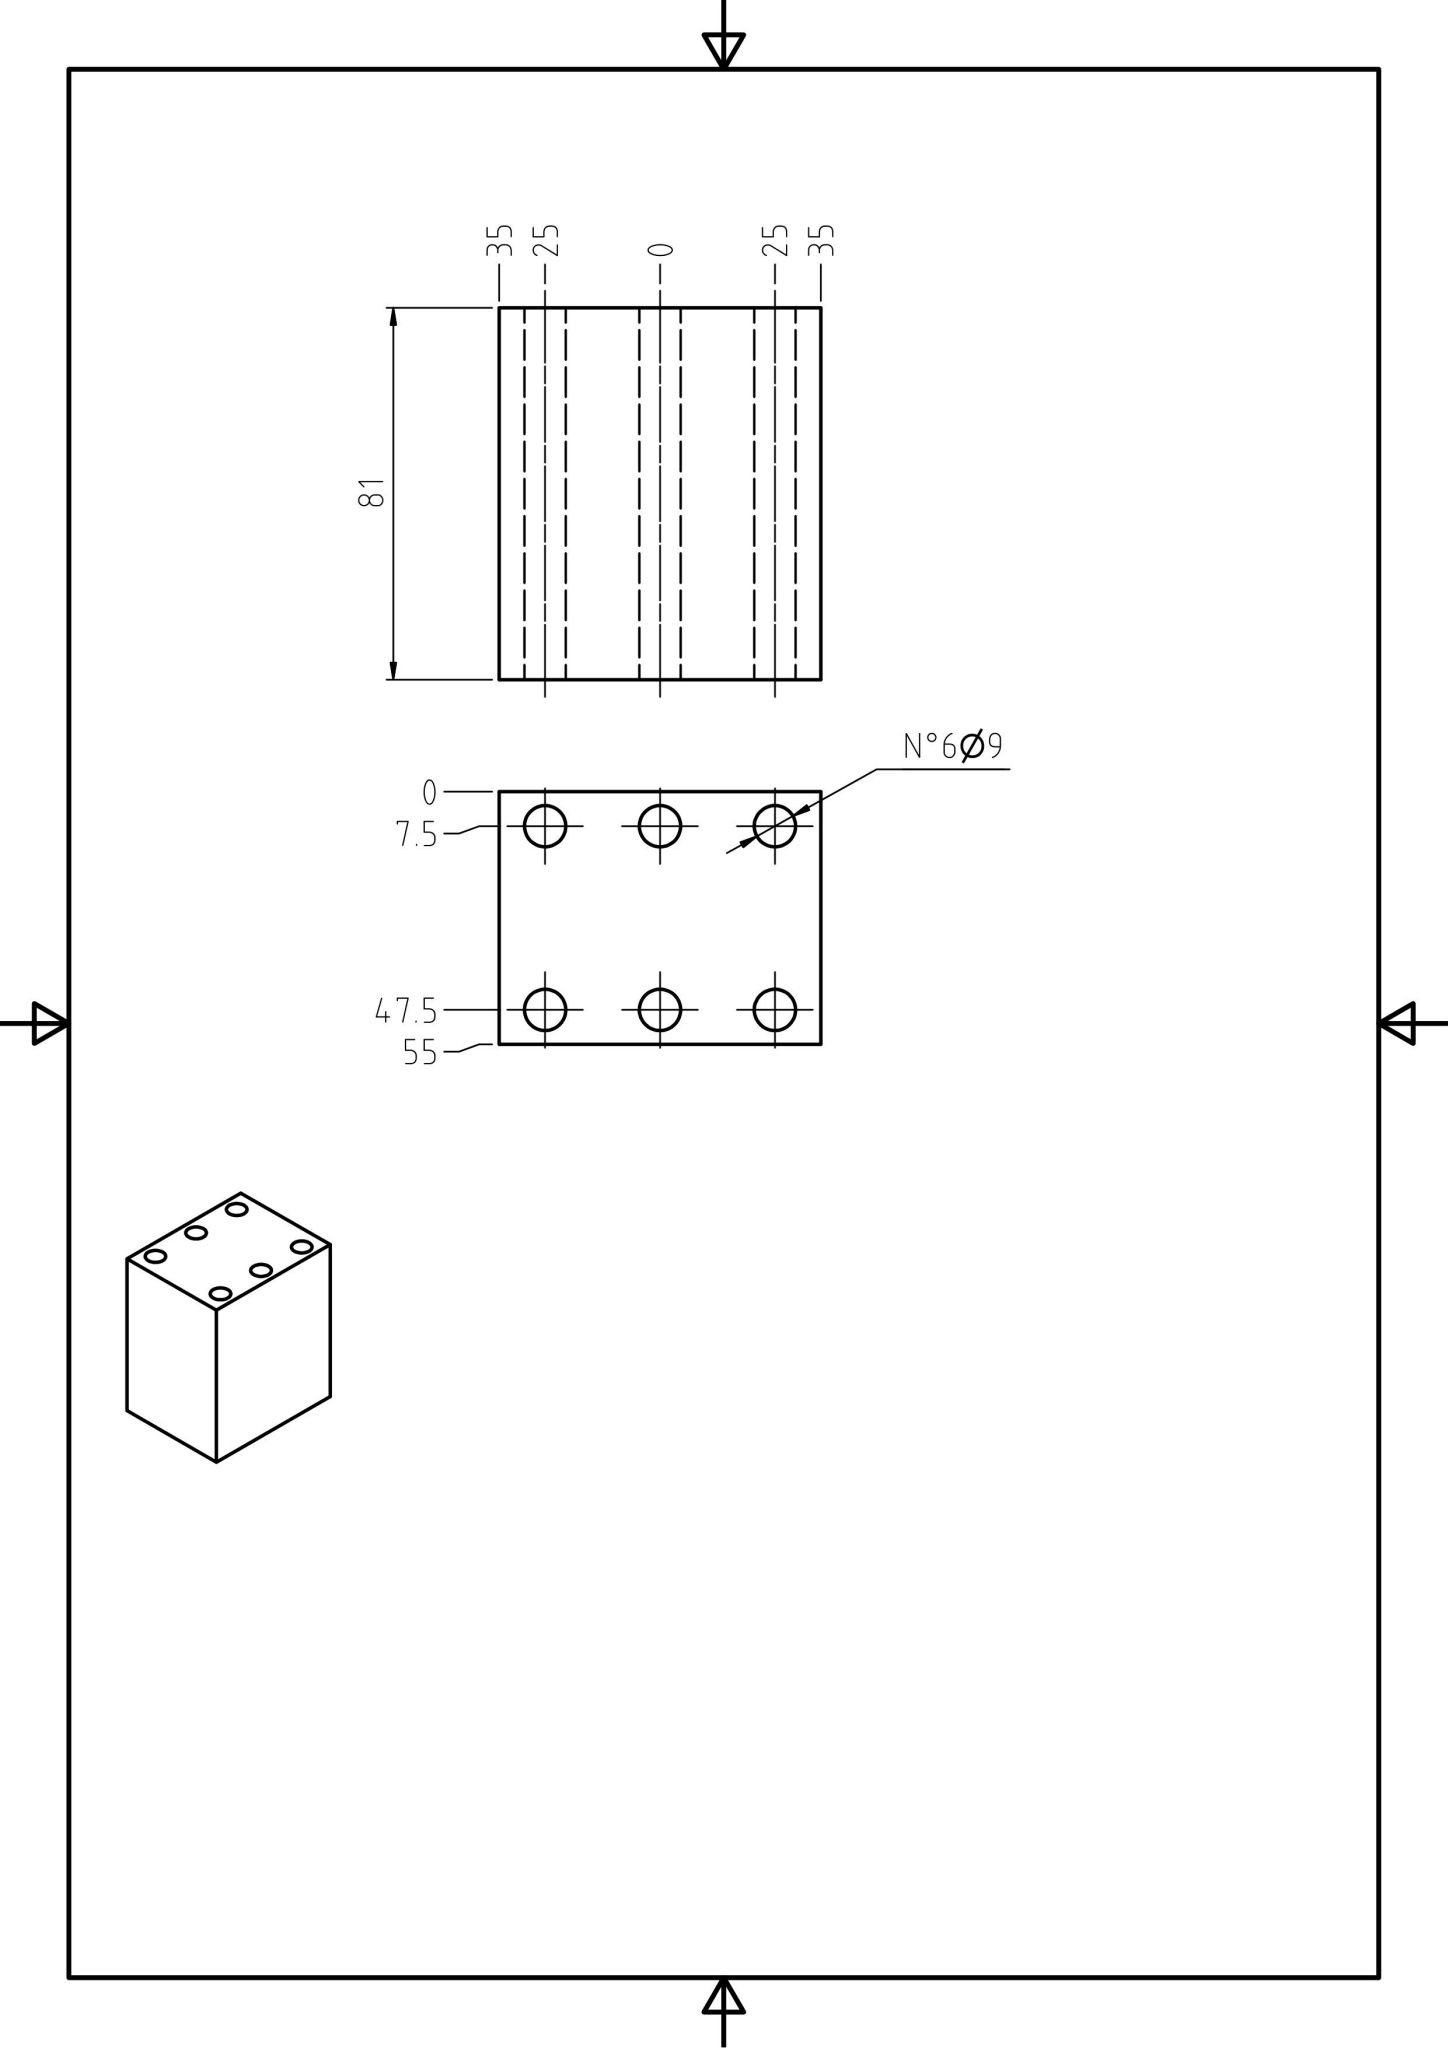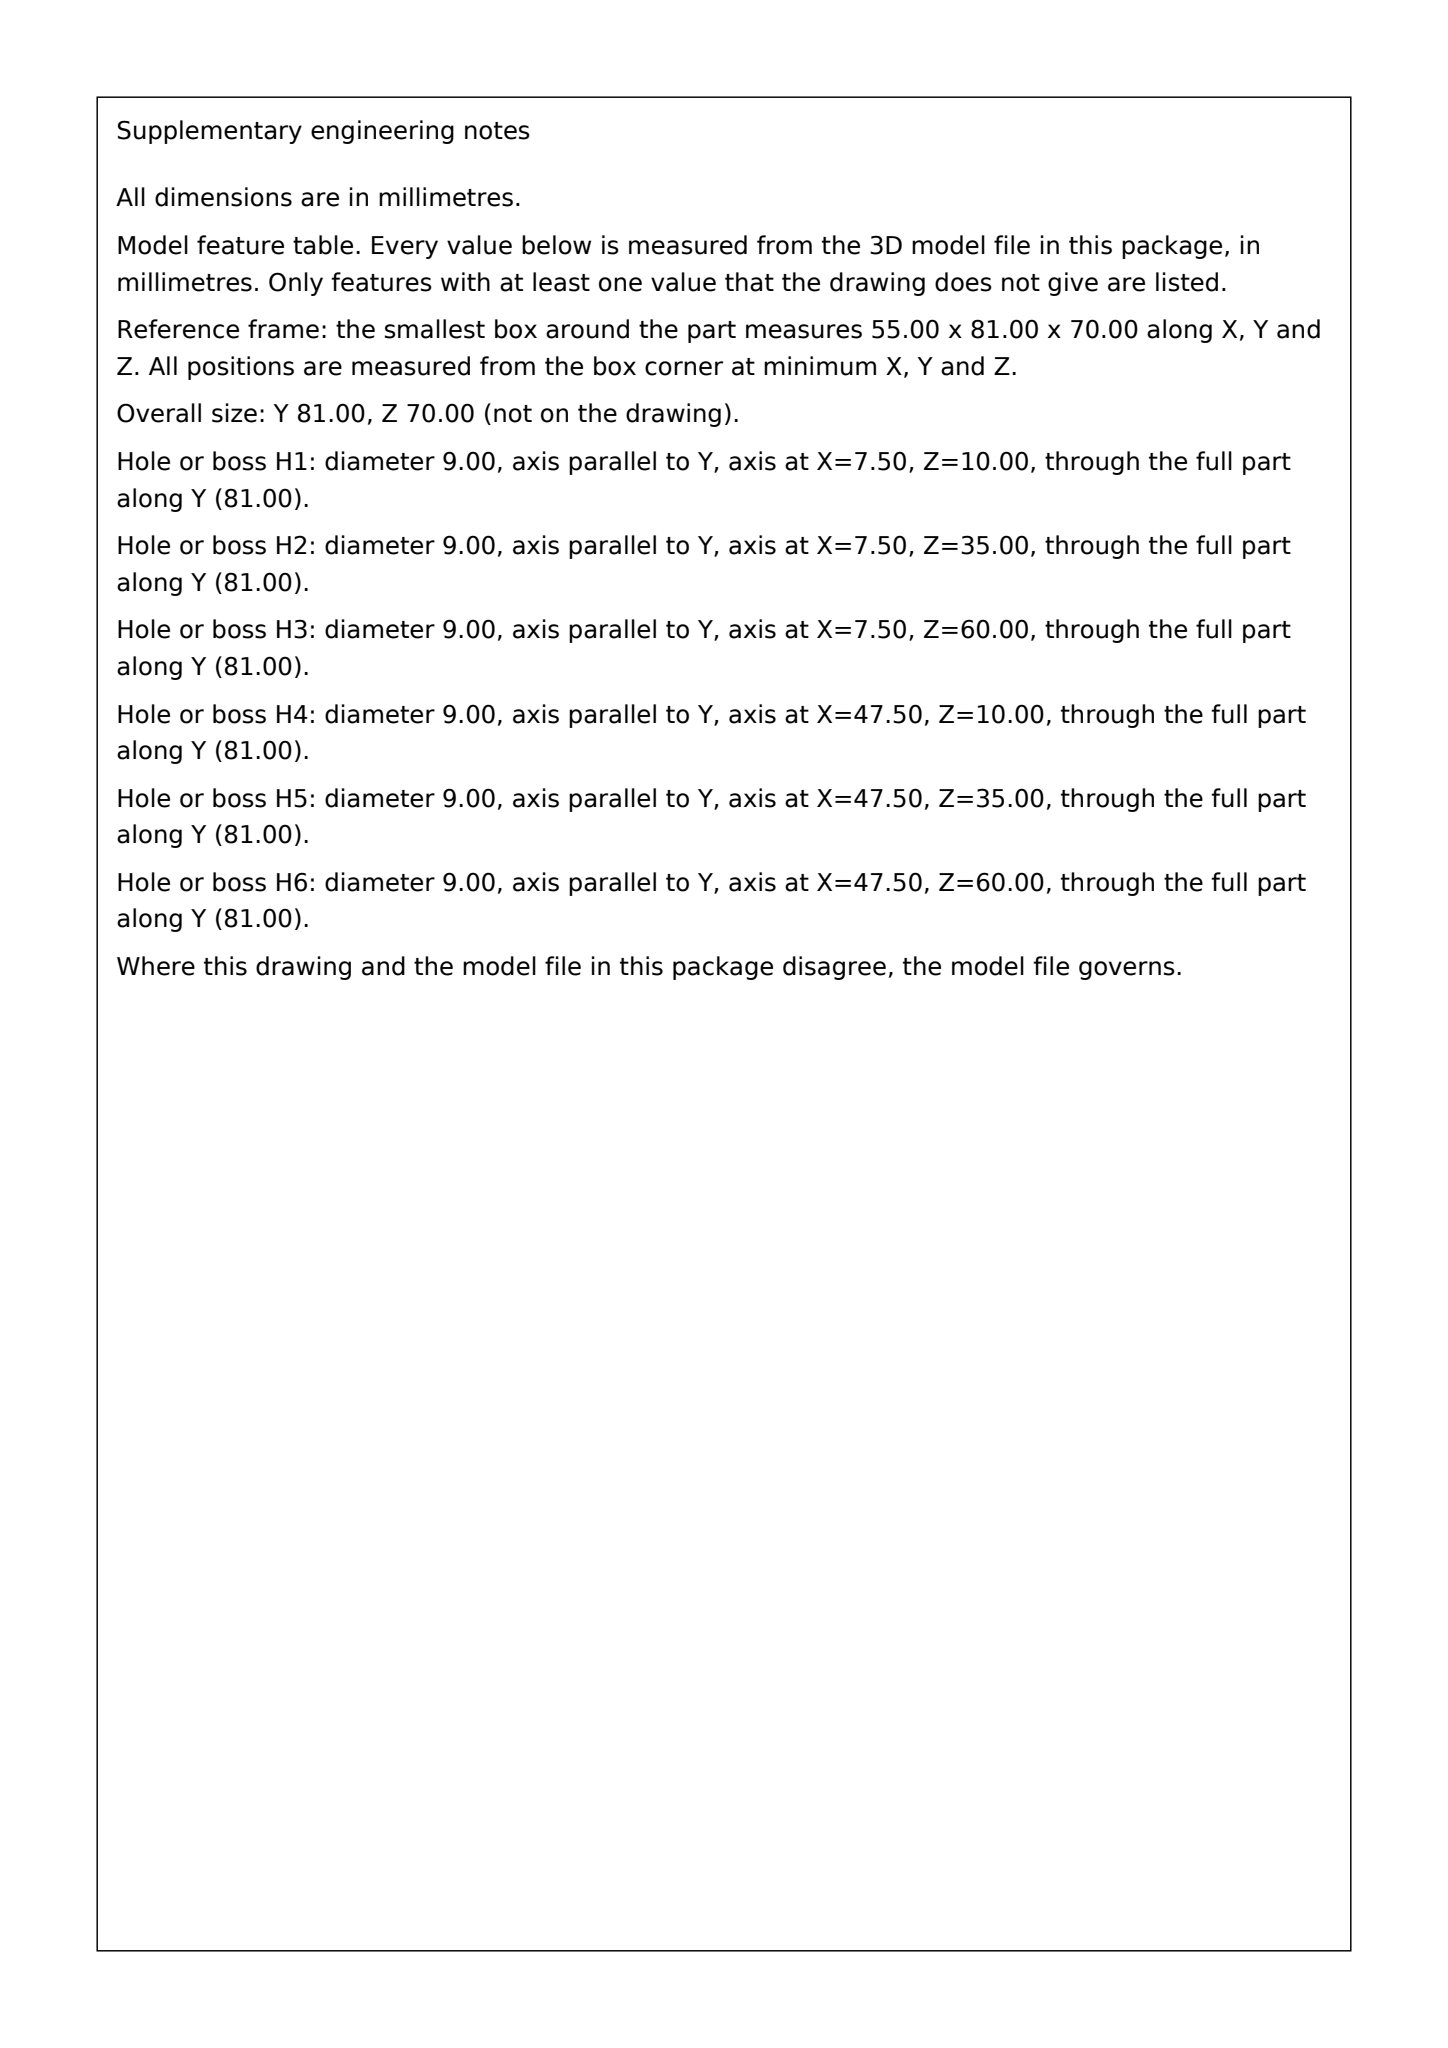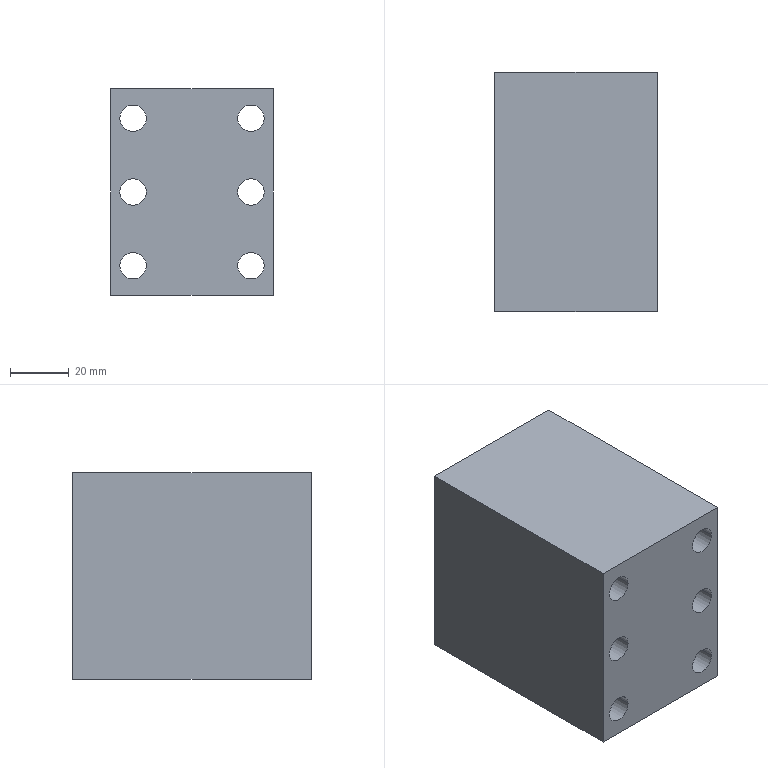Part | SolidWorks | mm | 1 solid | 18 faces | box 55 x 81 x 70 mm | volume 280932 mm3 | cylinder 12 | plane 6 | commonest cylinder face diameters 9 x12
STEP:
#1=CARTESIAN_POINT('',(15.5,81.,-25.));
#2=VERTEX_POINT('',#1);
#3=CARTESIAN_POINT('',(24.5,81.,-25.));
#4=VERTEX_POINT('',#3);
#5=CARTESIAN_POINT('',(20.,81.,-25.));
#6=DIRECTION('',(0.,-1.,0.));
#7=DIRECTION('',(1.,0.,0.));
#8=AXIS2_PLACEMENT_3D('',#5,#6,#7);
#9=CIRCLE('',#8,4.5);
#10=EDGE_CURVE('',#2,#4,#9,.T.);
#11=ORIENTED_EDGE('',*,*,#10,.F.);
#12=CARTESIAN_POINT('',(15.5,0.,-25.));
#13=VERTEX_POINT('',#12);
#14=CARTESIAN_POINT('',(15.5,120.358,-25.));
#15=DIRECTION('',(0.,-1.,0.));
#16=VECTOR('',#15,1000.);
#17=LINE('',#14,#16);
#18=EDGE_CURVE('',#2,#13,#17,.T.);
#19=ORIENTED_EDGE('',*,*,#18,.T.);
#20=CARTESIAN_POINT('',(24.5,0.,-25.));
#21=VERTEX_POINT('',#20);
#22=CARTESIAN_POINT('',(20.,0.,-25.));
#23=DIRECTION('',(0.,1.,0.));
#24=DIRECTION('',(1.,0.,0.));
#25=AXIS2_PLACEMENT_3D('',#22,#23,#24);
#26=CIRCLE('',#25,4.5);
#27=EDGE_CURVE('',#21,#13,#26,.T.);
#28=ORIENTED_EDGE('',*,*,#27,.F.);
#29=CARTESIAN_POINT('',(24.5,120.358,-25.));
#30=DIRECTION('',(0.,-1.,0.));
#31=VECTOR('',#30,1000.);
#32=LINE('',#29,#31);
#33=EDGE_CURVE('',#4,#21,#32,.T.);
#34=ORIENTED_EDGE('',*,*,#33,.F.);
#35=EDGE_LOOP('',(#11,#19,#28,#34));
#36=FACE_OUTER_BOUND('',#35,.T.);
#37=CARTESIAN_POINT('',(20.,120.358,-25.));
#38=DIRECTION('',(0.,-1.,0.));
#39=DIRECTION('',(1.,0.,0.));
#40=AXIS2_PLACEMENT_3D('',#37,#38,#39);
#41=CYLINDRICAL_SURFACE('',#40,4.5);
#42=ADVANCED_FACE('',(#36),#41,.F.);
#43=CARTESIAN_POINT('',(15.5,81.,25.));
#44=VERTEX_POINT('',#43);
#45=CARTESIAN_POINT('',(24.5,81.,25.));
#46=VERTEX_POINT('',#45);
#47=CARTESIAN_POINT('',(20.,81.,25.));
#48=DIRECTION('',(0.,-1.,0.));
#49=DIRECTION('',(1.,0.,0.));
#50=AXIS2_PLACEMENT_3D('',#47,#48,#49);
#51=CIRCLE('',#50,4.5);
#52=EDGE_CURVE('',#44,#46,#51,.T.);
#53=ORIENTED_EDGE('',*,*,#52,.F.);
#54=CARTESIAN_POINT('',(15.5,0.,25.));
#55=VERTEX_POINT('',#54);
#56=CARTESIAN_POINT('',(15.5,120.358,25.));
#57=DIRECTION('',(0.,-1.,0.));
#58=VECTOR('',#57,1000.);
#59=LINE('',#56,#58);
#60=EDGE_CURVE('',#44,#55,#59,.T.);
#61=ORIENTED_EDGE('',*,*,#60,.T.);
#62=CARTESIAN_POINT('',(24.5,0.,25.));
#63=VERTEX_POINT('',#62);
#64=CARTESIAN_POINT('',(20.,0.,25.));
#65=DIRECTION('',(0.,1.,0.));
#66=DIRECTION('',(1.,0.,0.));
#67=AXIS2_PLACEMENT_3D('',#64,#65,#66);
#68=CIRCLE('',#67,4.5);
#69=EDGE_CURVE('',#63,#55,#68,.T.);
#70=ORIENTED_EDGE('',*,*,#69,.F.);
#71=CARTESIAN_POINT('',(24.5,120.358,25.));
#72=DIRECTION('',(0.,-1.,0.));
#73=VECTOR('',#72,1000.);
#74=LINE('',#71,#73);
#75=EDGE_CURVE('',#46,#63,#74,.T.);
#76=ORIENTED_EDGE('',*,*,#75,.F.);
#77=EDGE_LOOP('',(#53,#61,#70,#76));
#78=FACE_OUTER_BOUND('',#77,.T.);
#79=CARTESIAN_POINT('',(20.,120.358,25.));
#80=DIRECTION('',(0.,-1.,0.));
#81=DIRECTION('',(1.,0.,0.));
#82=AXIS2_PLACEMENT_3D('',#79,#80,#81);
#83=CYLINDRICAL_SURFACE('',#82,4.5);
#84=ADVANCED_FACE('',(#78),#83,.F.);
#85=CARTESIAN_POINT('',(-24.5,81.,0.));
#86=VERTEX_POINT('',#85);
#87=CARTESIAN_POINT('',(-15.5,81.,0.));
#88=VERTEX_POINT('',#87);
#89=CARTESIAN_POINT('',(-20.,81.,0.));
#90=DIRECTION('',(0.,-1.,0.));
#91=DIRECTION('',(1.,0.,0.));
#92=AXIS2_PLACEMENT_3D('',#89,#90,#91);
#93=CIRCLE('',#92,4.5);
#94=EDGE_CURVE('',#86,#88,#93,.T.);
#95=ORIENTED_EDGE('',*,*,#94,.F.);
#96=CARTESIAN_POINT('',(-24.5,0.,0.));
#97=VERTEX_POINT('',#96);
#98=CARTESIAN_POINT('',(-24.5,120.358,0.));
#99=DIRECTION('',(0.,-1.,0.));
#100=VECTOR('',#99,1000.);
#101=LINE('',#98,#100);
#102=EDGE_CURVE('',#86,#97,#101,.T.);
#103=ORIENTED_EDGE('',*,*,#102,.T.);
#104=CARTESIAN_POINT('',(-15.5,0.,0.));
#105=VERTEX_POINT('',#104);
#106=CARTESIAN_POINT('',(-20.,0.,0.));
#107=DIRECTION('',(0.,1.,0.));
#108=DIRECTION('',(1.,0.,0.));
#109=AXIS2_PLACEMENT_3D('',#106,#107,#108);
#110=CIRCLE('',#109,4.5);
#111=EDGE_CURVE('',#105,#97,#110,.T.);
#112=ORIENTED_EDGE('',*,*,#111,.F.);
#113=CARTESIAN_POINT('',(-15.5,120.358,0.));
#114=DIRECTION('',(0.,-1.,0.));
#115=VECTOR('',#114,1000.);
#116=LINE('',#113,#115);
#117=EDGE_CURVE('',#88,#105,#116,.T.);
#118=ORIENTED_EDGE('',*,*,#117,.F.);
#119=EDGE_LOOP('',(#95,#103,#112,#118));
#120=FACE_OUTER_BOUND('',#119,.T.);
#121=CARTESIAN_POINT('',(-20.,120.358,0.));
#122=DIRECTION('',(0.,-1.,0.));
#123=DIRECTION('',(1.,0.,0.));
#124=AXIS2_PLACEMENT_3D('',#121,#122,#123);
#125=CYLINDRICAL_SURFACE('',#124,4.5);
#126=ADVANCED_FACE('',(#120),#125,.F.);
#127=CARTESIAN_POINT('',(-24.5,81.,25.));
#128=VERTEX_POINT('',#127);
#129=CARTESIAN_POINT('',(-15.5,81.,25.));
#130=VERTEX_POINT('',#129);
#131=CARTESIAN_POINT('',(-20.,81.,25.));
#132=DIRECTION('',(0.,-1.,0.));
#133=DIRECTION('',(1.,0.,0.));
#134=AXIS2_PLACEMENT_3D('',#131,#132,#133);
#135=CIRCLE('',#134,4.5);
#136=EDGE_CURVE('',#128,#130,#135,.T.);
#137=ORIENTED_EDGE('',*,*,#136,.F.);
#138=CARTESIAN_POINT('',(-24.5,0.,25.));
#139=VERTEX_POINT('',#138);
#140=CARTESIAN_POINT('',(-24.5,120.358,25.));
#141=DIRECTION('',(0.,-1.,0.));
#142=VECTOR('',#141,1000.);
#143=LINE('',#140,#142);
#144=EDGE_CURVE('',#128,#139,#143,.T.);
#145=ORIENTED_EDGE('',*,*,#144,.T.);
#146=CARTESIAN_POINT('',(-15.5,0.,25.));
#147=VERTEX_POINT('',#146);
#148=CARTESIAN_POINT('',(-20.,0.,25.));
#149=DIRECTION('',(0.,1.,0.));
#150=DIRECTION('',(1.,0.,0.));
#151=AXIS2_PLACEMENT_3D('',#148,#149,#150);
#152=CIRCLE('',#151,4.5);
#153=EDGE_CURVE('',#147,#139,#152,.T.);
#154=ORIENTED_EDGE('',*,*,#153,.F.);
#155=CARTESIAN_POINT('',(-15.5,120.358,25.));
#156=DIRECTION('',(0.,-1.,0.));
#157=VECTOR('',#156,1000.);
#158=LINE('',#155,#157);
#159=EDGE_CURVE('',#130,#147,#158,.T.);
#160=ORIENTED_EDGE('',*,*,#159,.F.);
#161=EDGE_LOOP('',(#137,#145,#154,#160));
#162=FACE_OUTER_BOUND('',#161,.T.);
#163=CARTESIAN_POINT('',(-20.,120.358,25.));
#164=DIRECTION('',(0.,-1.,0.));
#165=DIRECTION('',(1.,0.,0.));
#166=AXIS2_PLACEMENT_3D('',#163,#164,#165);
#167=CYLINDRICAL_SURFACE('',#166,4.5);
#168=ADVANCED_FACE('',(#162),#167,.F.);
#169=CARTESIAN_POINT('',(-24.5,81.,-25.));
#170=VERTEX_POINT('',#169);
#171=CARTESIAN_POINT('',(-15.5,81.,-25.));
#172=VERTEX_POINT('',#171);
#173=CARTESIAN_POINT('',(-20.,81.,-25.));
#174=DIRECTION('',(0.,-1.,0.));
#175=DIRECTION('',(1.,0.,0.));
#176=AXIS2_PLACEMENT_3D('',#173,#174,#175);
#177=CIRCLE('',#176,4.5);
#178=EDGE_CURVE('',#170,#172,#177,.T.);
#179=ORIENTED_EDGE('',*,*,#178,.F.);
#180=CARTESIAN_POINT('',(-24.5,0.,-25.));
#181=VERTEX_POINT('',#180);
#182=CARTESIAN_POINT('',(-24.5,120.358,-25.));
#183=DIRECTION('',(0.,-1.,0.));
#184=VECTOR('',#183,1000.);
#185=LINE('',#182,#184);
#186=EDGE_CURVE('',#170,#181,#185,.T.);
#187=ORIENTED_EDGE('',*,*,#186,.T.);
#188=CARTESIAN_POINT('',(-15.5,0.,-25.));
#189=VERTEX_POINT('',#188);
#190=CARTESIAN_POINT('',(-20.,0.,-25.));
#191=DIRECTION('',(0.,1.,0.));
#192=DIRECTION('',(1.,0.,0.));
#193=AXIS2_PLACEMENT_3D('',#190,#191,#192);
#194=CIRCLE('',#193,4.5);
#195=EDGE_CURVE('',#189,#181,#194,.T.);
#196=ORIENTED_EDGE('',*,*,#195,.F.);
#197=CARTESIAN_POINT('',(-15.5,120.358,-25.));
#198=DIRECTION('',(0.,-1.,0.));
#199=VECTOR('',#198,1000.);
#200=LINE('',#197,#199);
#201=EDGE_CURVE('',#172,#189,#200,.T.);
#202=ORIENTED_EDGE('',*,*,#201,.F.);
#203=EDGE_LOOP('',(#179,#187,#196,#202));
#204=FACE_OUTER_BOUND('',#203,.T.);
#205=CARTESIAN_POINT('',(-20.,120.358,-25.));
#206=DIRECTION('',(0.,-1.,0.));
#207=DIRECTION('',(1.,0.,0.));
#208=AXIS2_PLACEMENT_3D('',#205,#206,#207);
#209=CYLINDRICAL_SURFACE('',#208,4.5);
#210=ADVANCED_FACE('',(#204),#209,.F.);
#211=CARTESIAN_POINT('',(15.5,81.,0.));
#212=VERTEX_POINT('',#211);
#213=CARTESIAN_POINT('',(24.5,81.,0.));
#214=VERTEX_POINT('',#213);
#215=CARTESIAN_POINT('',(20.,81.,0.));
#216=DIRECTION('',(0.,-1.,0.));
#217=DIRECTION('',(1.,0.,0.));
#218=AXIS2_PLACEMENT_3D('',#215,#216,#217);
#219=CIRCLE('',#218,4.5);
#220=EDGE_CURVE('',#212,#214,#219,.T.);
#221=ORIENTED_EDGE('',*,*,#220,.F.);
#222=CARTESIAN_POINT('',(15.5,0.,0.));
#223=VERTEX_POINT('',#222);
#224=CARTESIAN_POINT('',(15.5,120.358,0.));
#225=DIRECTION('',(0.,-1.,0.));
#226=VECTOR('',#225,1000.);
#227=LINE('',#224,#226);
#228=EDGE_CURVE('',#212,#223,#227,.T.);
#229=ORIENTED_EDGE('',*,*,#228,.T.);
#230=CARTESIAN_POINT('',(24.5,0.,0.));
#231=VERTEX_POINT('',#230);
#232=CARTESIAN_POINT('',(20.,0.,0.));
#233=DIRECTION('',(0.,1.,0.));
#234=DIRECTION('',(1.,0.,0.));
#235=AXIS2_PLACEMENT_3D('',#232,#233,#234);
#236=CIRCLE('',#235,4.5);
#237=EDGE_CURVE('',#231,#223,#236,.T.);
#238=ORIENTED_EDGE('',*,*,#237,.F.);
#239=CARTESIAN_POINT('',(24.5,120.358,0.));
#240=DIRECTION('',(0.,-1.,0.));
#241=VECTOR('',#240,1000.);
#242=LINE('',#239,#241);
#243=EDGE_CURVE('',#214,#231,#242,.T.);
#244=ORIENTED_EDGE('',*,*,#243,.F.);
#245=EDGE_LOOP('',(#221,#229,#238,#244));
#246=FACE_OUTER_BOUND('',#245,.T.);
#247=CARTESIAN_POINT('',(20.,120.358,0.));
#248=DIRECTION('',(0.,-1.,0.));
#249=DIRECTION('',(1.,0.,0.));
#250=AXIS2_PLACEMENT_3D('',#247,#248,#249);
#251=CYLINDRICAL_SURFACE('',#250,4.5);
#252=ADVANCED_FACE('',(#246),#251,.F.);
#253=ORIENTED_EDGE('',*,*,#228,.F.);
#254=CARTESIAN_POINT('',(20.,81.,0.));
#255=DIRECTION('',(0.,-1.,0.));
#256=DIRECTION('',(1.,0.,0.));
#257=AXIS2_PLACEMENT_3D('',#254,#255,#256);
#258=CIRCLE('',#257,4.5);
#259=EDGE_CURVE('',#214,#212,#258,.T.);
#260=ORIENTED_EDGE('',*,*,#259,.F.);
#261=ORIENTED_EDGE('',*,*,#243,.T.);
#262=CARTESIAN_POINT('',(20.,0.,0.));
#263=DIRECTION('',(0.,1.,0.));
#264=DIRECTION('',(1.,0.,0.));
#265=AXIS2_PLACEMENT_3D('',#262,#263,#264);
#266=CIRCLE('',#265,4.5);
#267=EDGE_CURVE('',#223,#231,#266,.T.);
#268=ORIENTED_EDGE('',*,*,#267,.F.);
#269=EDGE_LOOP('',(#253,#260,#261,#268));
#270=FACE_OUTER_BOUND('',#269,.T.);
#271=CARTESIAN_POINT('',(20.,120.358,0.));
#272=DIRECTION('',(0.,-1.,0.));
#273=DIRECTION('',(1.,0.,0.));
#274=AXIS2_PLACEMENT_3D('',#271,#272,#273);
#275=CYLINDRICAL_SURFACE('',#274,4.5);
#276=ADVANCED_FACE('',(#270),#275,.F.);
#277=ORIENTED_EDGE('',*,*,#186,.F.);
#278=CARTESIAN_POINT('',(-20.,81.,-25.));
#279=DIRECTION('',(0.,-1.,0.));
#280=DIRECTION('',(1.,0.,0.));
#281=AXIS2_PLACEMENT_3D('',#278,#279,#280);
#282=CIRCLE('',#281,4.5);
#283=EDGE_CURVE('',#172,#170,#282,.T.);
#284=ORIENTED_EDGE('',*,*,#283,.F.);
#285=ORIENTED_EDGE('',*,*,#201,.T.);
#286=CARTESIAN_POINT('',(-20.,0.,-25.));
#287=DIRECTION('',(0.,1.,0.));
#288=DIRECTION('',(1.,0.,0.));
#289=AXIS2_PLACEMENT_3D('',#286,#287,#288);
#290=CIRCLE('',#289,4.5);
#291=EDGE_CURVE('',#181,#189,#290,.T.);
#292=ORIENTED_EDGE('',*,*,#291,.F.);
#293=EDGE_LOOP('',(#277,#284,#285,#292));
#294=FACE_OUTER_BOUND('',#293,.T.);
#295=CARTESIAN_POINT('',(-20.,120.358,-25.));
#296=DIRECTION('',(0.,-1.,0.));
#297=DIRECTION('',(1.,0.,0.));
#298=AXIS2_PLACEMENT_3D('',#295,#296,#297);
#299=CYLINDRICAL_SURFACE('',#298,4.5);
#300=ADVANCED_FACE('',(#294),#299,.F.);
#301=ORIENTED_EDGE('',*,*,#144,.F.);
#302=CARTESIAN_POINT('',(-20.,81.,25.));
#303=DIRECTION('',(0.,-1.,0.));
#304=DIRECTION('',(1.,0.,0.));
#305=AXIS2_PLACEMENT_3D('',#302,#303,#304);
#306=CIRCLE('',#305,4.5);
#307=EDGE_CURVE('',#130,#128,#306,.T.);
#308=ORIENTED_EDGE('',*,*,#307,.F.);
#309=ORIENTED_EDGE('',*,*,#159,.T.);
#310=CARTESIAN_POINT('',(-20.,0.,25.));
#311=DIRECTION('',(0.,1.,0.));
#312=DIRECTION('',(1.,0.,0.));
#313=AXIS2_PLACEMENT_3D('',#310,#311,#312);
#314=CIRCLE('',#313,4.5);
#315=EDGE_CURVE('',#139,#147,#314,.T.);
#316=ORIENTED_EDGE('',*,*,#315,.F.);
#317=EDGE_LOOP('',(#301,#308,#309,#316));
#318=FACE_OUTER_BOUND('',#317,.T.);
#319=CARTESIAN_POINT('',(-20.,120.358,25.));
#320=DIRECTION('',(0.,-1.,0.));
#321=DIRECTION('',(1.,0.,0.));
#322=AXIS2_PLACEMENT_3D('',#319,#320,#321);
#323=CYLINDRICAL_SURFACE('',#322,4.5);
#324=ADVANCED_FACE('',(#318),#323,.F.);
#325=ORIENTED_EDGE('',*,*,#102,.F.);
#326=CARTESIAN_POINT('',(-20.,81.,0.));
#327=DIRECTION('',(0.,-1.,0.));
#328=DIRECTION('',(1.,0.,0.));
#329=AXIS2_PLACEMENT_3D('',#326,#327,#328);
#330=CIRCLE('',#329,4.5);
#331=EDGE_CURVE('',#88,#86,#330,.T.);
#332=ORIENTED_EDGE('',*,*,#331,.F.);
#333=ORIENTED_EDGE('',*,*,#117,.T.);
#334=CARTESIAN_POINT('',(-20.,0.,0.));
#335=DIRECTION('',(0.,1.,0.));
#336=DIRECTION('',(1.,0.,0.));
#337=AXIS2_PLACEMENT_3D('',#334,#335,#336);
#338=CIRCLE('',#337,4.5);
#339=EDGE_CURVE('',#97,#105,#338,.T.);
#340=ORIENTED_EDGE('',*,*,#339,.F.);
#341=EDGE_LOOP('',(#325,#332,#333,#340));
#342=FACE_OUTER_BOUND('',#341,.T.);
#343=CARTESIAN_POINT('',(-20.,120.358,0.));
#344=DIRECTION('',(0.,-1.,0.));
#345=DIRECTION('',(1.,0.,0.));
#346=AXIS2_PLACEMENT_3D('',#343,#344,#345);
#347=CYLINDRICAL_SURFACE('',#346,4.5);
#348=ADVANCED_FACE('',(#342),#347,.F.);
#349=ORIENTED_EDGE('',*,*,#60,.F.);
#350=CARTESIAN_POINT('',(20.,81.,25.));
#351=DIRECTION('',(0.,-1.,0.));
#352=DIRECTION('',(1.,0.,0.));
#353=AXIS2_PLACEMENT_3D('',#350,#351,#352);
#354=CIRCLE('',#353,4.5);
#355=EDGE_CURVE('',#46,#44,#354,.T.);
#356=ORIENTED_EDGE('',*,*,#355,.F.);
#357=ORIENTED_EDGE('',*,*,#75,.T.);
#358=CARTESIAN_POINT('',(20.,0.,25.));
#359=DIRECTION('',(0.,1.,0.));
#360=DIRECTION('',(1.,0.,0.));
#361=AXIS2_PLACEMENT_3D('',#358,#359,#360);
#362=CIRCLE('',#361,4.5);
#363=EDGE_CURVE('',#55,#63,#362,.T.);
#364=ORIENTED_EDGE('',*,*,#363,.F.);
#365=EDGE_LOOP('',(#349,#356,#357,#364));
#366=FACE_OUTER_BOUND('',#365,.T.);
#367=CARTESIAN_POINT('',(20.,120.358,25.));
#368=DIRECTION('',(0.,-1.,0.));
#369=DIRECTION('',(1.,0.,0.));
#370=AXIS2_PLACEMENT_3D('',#367,#368,#369);
#371=CYLINDRICAL_SURFACE('',#370,4.5);
#372=ADVANCED_FACE('',(#366),#371,.F.);
#373=ORIENTED_EDGE('',*,*,#18,.F.);
#374=CARTESIAN_POINT('',(20.,81.,-25.));
#375=DIRECTION('',(0.,-1.,0.));
#376=DIRECTION('',(1.,0.,0.));
#377=AXIS2_PLACEMENT_3D('',#374,#375,#376);
#378=CIRCLE('',#377,4.5);
#379=EDGE_CURVE('',#4,#2,#378,.T.);
#380=ORIENTED_EDGE('',*,*,#379,.F.);
#381=ORIENTED_EDGE('',*,*,#33,.T.);
#382=CARTESIAN_POINT('',(20.,0.,-25.));
#383=DIRECTION('',(0.,1.,0.));
#384=DIRECTION('',(1.,0.,0.));
#385=AXIS2_PLACEMENT_3D('',#382,#383,#384);
#386=CIRCLE('',#385,4.5);
#387=EDGE_CURVE('',#13,#21,#386,.T.);
#388=ORIENTED_EDGE('',*,*,#387,.F.);
#389=EDGE_LOOP('',(#373,#380,#381,#388));
#390=FACE_OUTER_BOUND('',#389,.T.);
#391=CARTESIAN_POINT('',(20.,120.358,-25.));
#392=DIRECTION('',(0.,-1.,0.));
#393=DIRECTION('',(1.,0.,0.));
#394=AXIS2_PLACEMENT_3D('',#391,#392,#393);
#395=CYLINDRICAL_SURFACE('',#394,4.5);
#396=ADVANCED_FACE('',(#390),#395,.F.);
#397=CARTESIAN_POINT('',(-27.5,0.,35.));
#398=VERTEX_POINT('',#397);
#399=CARTESIAN_POINT('',(27.5,0.,35.));
#400=VERTEX_POINT('',#399);
#401=CARTESIAN_POINT('',(-27.5,0.,35.));
#402=DIRECTION('',(1.,0.,0.));
#403=VECTOR('',#402,1000.);
#404=LINE('',#401,#403);
#405=EDGE_CURVE('',#398,#400,#404,.T.);
#406=ORIENTED_EDGE('',*,*,#405,.T.);
#407=CARTESIAN_POINT('',(27.5,81.,35.));
#408=VERTEX_POINT('',#407);
#409=CARTESIAN_POINT('',(27.5,0.,35.));
#410=DIRECTION('',(0.,1.,0.));
#411=VECTOR('',#410,1000.);
#412=LINE('',#409,#411);
#413=EDGE_CURVE('',#400,#408,#412,.T.);
#414=ORIENTED_EDGE('',*,*,#413,.T.);
#415=CARTESIAN_POINT('',(-27.5,81.,35.));
#416=VERTEX_POINT('',#415);
#417=CARTESIAN_POINT('',(-27.5,81.,35.));
#418=DIRECTION('',(1.,0.,0.));
#419=VECTOR('',#418,1000.);
#420=LINE('',#417,#419);
#421=EDGE_CURVE('',#416,#408,#420,.T.);
#422=ORIENTED_EDGE('',*,*,#421,.F.);
#423=CARTESIAN_POINT('',(-27.5,0.,35.));
#424=DIRECTION('',(0.,1.,0.));
#425=VECTOR('',#424,1000.);
#426=LINE('',#423,#425);
#427=EDGE_CURVE('',#398,#416,#426,.T.);
#428=ORIENTED_EDGE('',*,*,#427,.F.);
#429=EDGE_LOOP('',(#406,#414,#422,#428));
#430=FACE_OUTER_BOUND('',#429,.T.);
#431=CARTESIAN_POINT('',(-27.5,0.,35.));
#432=DIRECTION('',(0.,0.,1.));
#433=DIRECTION('',(1.,0.,0.));
#434=AXIS2_PLACEMENT_3D('',#431,#432,#433);
#435=PLANE('',#434);
#436=ADVANCED_FACE('',(#430),#435,.T.);
#437=CARTESIAN_POINT('',(-27.5,0.,-35.));
#438=VERTEX_POINT('',#437);
#439=CARTESIAN_POINT('',(-27.5,0.,-35.));
#440=DIRECTION('',(0.,0.,1.));
#441=VECTOR('',#440,1000.);
#442=LINE('',#439,#441);
#443=EDGE_CURVE('',#438,#398,#442,.T.);
#444=ORIENTED_EDGE('',*,*,#443,.T.);
#445=ORIENTED_EDGE('',*,*,#427,.T.);
#446=CARTESIAN_POINT('',(-27.5,81.,-35.));
#447=VERTEX_POINT('',#446);
#448=CARTESIAN_POINT('',(-27.5,81.,-35.));
#449=DIRECTION('',(0.,0.,1.));
#450=VECTOR('',#449,1000.);
#451=LINE('',#448,#450);
#452=EDGE_CURVE('',#447,#416,#451,.T.);
#453=ORIENTED_EDGE('',*,*,#452,.F.);
#454=CARTESIAN_POINT('',(-27.5,0.,-35.));
#455=DIRECTION('',(0.,1.,0.));
#456=VECTOR('',#455,1000.);
#457=LINE('',#454,#456);
#458=EDGE_CURVE('',#438,#447,#457,.T.);
#459=ORIENTED_EDGE('',*,*,#458,.F.);
#460=EDGE_LOOP('',(#444,#445,#453,#459));
#461=FACE_OUTER_BOUND('',#460,.T.);
#462=CARTESIAN_POINT('',(-27.5,0.,-35.));
#463=DIRECTION('',(-1.,0.,0.));
#464=DIRECTION('',(0.,0.,1.));
#465=AXIS2_PLACEMENT_3D('',#462,#463,#464);
#466=PLANE('',#465);
#467=ADVANCED_FACE('',(#461),#466,.T.);
#468=CARTESIAN_POINT('',(27.5,0.,-35.));
#469=VERTEX_POINT('',#468);
#470=CARTESIAN_POINT('',(27.5,0.,-35.));
#471=DIRECTION('',(-1.,0.,0.));
#472=VECTOR('',#471,1000.);
#473=LINE('',#470,#472);
#474=EDGE_CURVE('',#469,#438,#473,.T.);
#475=ORIENTED_EDGE('',*,*,#474,.T.);
#476=ORIENTED_EDGE('',*,*,#458,.T.);
#477=CARTESIAN_POINT('',(27.5,81.,-35.));
#478=VERTEX_POINT('',#477);
#479=CARTESIAN_POINT('',(27.5,81.,-35.));
#480=DIRECTION('',(-1.,0.,0.));
#481=VECTOR('',#480,1000.);
#482=LINE('',#479,#481);
#483=EDGE_CURVE('',#478,#447,#482,.T.);
#484=ORIENTED_EDGE('',*,*,#483,.F.);
#485=CARTESIAN_POINT('',(27.5,0.,-35.));
#486=DIRECTION('',(0.,1.,0.));
#487=VECTOR('',#486,1000.);
#488=LINE('',#485,#487);
#489=EDGE_CURVE('',#469,#478,#488,.T.);
#490=ORIENTED_EDGE('',*,*,#489,.F.);
#491=EDGE_LOOP('',(#475,#476,#484,#490));
#492=FACE_OUTER_BOUND('',#491,.T.);
#493=CARTESIAN_POINT('',(27.5,0.,-35.));
#494=DIRECTION('',(0.,0.,-1.));
#495=DIRECTION('',(0.,-1.,0.));
#496=AXIS2_PLACEMENT_3D('',#493,#494,#495);
#497=PLANE('',#496);
#498=ADVANCED_FACE('',(#492),#497,.T.);
#499=CARTESIAN_POINT('',(27.5,0.,35.));
#500=DIRECTION('',(0.,0.,-1.));
#501=VECTOR('',#500,1000.);
#502=LINE('',#499,#501);
#503=EDGE_CURVE('',#400,#469,#502,.T.);
#504=ORIENTED_EDGE('',*,*,#503,.T.);
#505=ORIENTED_EDGE('',*,*,#489,.T.);
#506=CARTESIAN_POINT('',(27.5,81.,35.));
#507=DIRECTION('',(0.,0.,-1.));
#508=VECTOR('',#507,1000.);
#509=LINE('',#506,#508);
#510=EDGE_CURVE('',#408,#478,#509,.T.);
#511=ORIENTED_EDGE('',*,*,#510,.F.);
#512=ORIENTED_EDGE('',*,*,#413,.F.);
#513=EDGE_LOOP('',(#504,#505,#511,#512));
#514=FACE_OUTER_BOUND('',#513,.T.);
#515=CARTESIAN_POINT('',(27.5,0.,35.));
#516=DIRECTION('',(1.,0.,0.));
#517=DIRECTION('',(0.,1.,0.));
#518=AXIS2_PLACEMENT_3D('',#515,#516,#517);
#519=PLANE('',#518);
#520=ADVANCED_FACE('',(#514),#519,.T.);
#521=ORIENTED_EDGE('',*,*,#510,.T.);
#522=ORIENTED_EDGE('',*,*,#483,.T.);
#523=ORIENTED_EDGE('',*,*,#452,.T.);
#524=ORIENTED_EDGE('',*,*,#421,.T.);
#525=EDGE_LOOP('',(#521,#522,#523,#524));
#526=FACE_OUTER_BOUND('',#525,.T.);
#527=ORIENTED_EDGE('',*,*,#259,.T.);
#528=ORIENTED_EDGE('',*,*,#220,.T.);
#529=EDGE_LOOP('',(#527,#528));
#530=FACE_BOUND('',#529,.T.);
#531=ORIENTED_EDGE('',*,*,#283,.T.);
#532=ORIENTED_EDGE('',*,*,#178,.T.);
#533=EDGE_LOOP('',(#531,#532));
#534=FACE_BOUND('',#533,.T.);
#535=ORIENTED_EDGE('',*,*,#307,.T.);
#536=ORIENTED_EDGE('',*,*,#136,.T.);
#537=EDGE_LOOP('',(#535,#536));
#538=FACE_BOUND('',#537,.T.);
#539=ORIENTED_EDGE('',*,*,#331,.T.);
#540=ORIENTED_EDGE('',*,*,#94,.T.);
#541=EDGE_LOOP('',(#539,#540));
#542=FACE_BOUND('',#541,.T.);
#543=ORIENTED_EDGE('',*,*,#355,.T.);
#544=ORIENTED_EDGE('',*,*,#52,.T.);
#545=EDGE_LOOP('',(#543,#544));
#546=FACE_BOUND('',#545,.T.);
#547=ORIENTED_EDGE('',*,*,#379,.T.);
#548=ORIENTED_EDGE('',*,*,#10,.T.);
#549=EDGE_LOOP('',(#547,#548));
#550=FACE_BOUND('',#549,.T.);
#551=CARTESIAN_POINT('',(0.,81.,0.));
#552=DIRECTION('',(0.,1.,0.));
#553=DIRECTION('',(1.,0.,0.));
#554=AXIS2_PLACEMENT_3D('',#551,#552,#553);
#555=PLANE('',#554);
#556=ADVANCED_FACE('',(#526,#530,#534,#538,#542,#546,#550),#555,.T.);
#557=ORIENTED_EDGE('',*,*,#503,.F.);
#558=ORIENTED_EDGE('',*,*,#405,.F.);
#559=ORIENTED_EDGE('',*,*,#443,.F.);
#560=ORIENTED_EDGE('',*,*,#474,.F.);
#561=EDGE_LOOP('',(#557,#558,#559,#560));
#562=FACE_OUTER_BOUND('',#561,.T.);
#563=ORIENTED_EDGE('',*,*,#237,.T.);
#564=ORIENTED_EDGE('',*,*,#267,.T.);
#565=EDGE_LOOP('',(#563,#564));
#566=FACE_BOUND('',#565,.T.);
#567=ORIENTED_EDGE('',*,*,#195,.T.);
#568=ORIENTED_EDGE('',*,*,#291,.T.);
#569=EDGE_LOOP('',(#567,#568));
#570=FACE_BOUND('',#569,.T.);
#571=ORIENTED_EDGE('',*,*,#153,.T.);
#572=ORIENTED_EDGE('',*,*,#315,.T.);
#573=EDGE_LOOP('',(#571,#572));
#574=FACE_BOUND('',#573,.T.);
#575=ORIENTED_EDGE('',*,*,#111,.T.);
#576=ORIENTED_EDGE('',*,*,#339,.T.);
#577=EDGE_LOOP('',(#575,#576));
#578=FACE_BOUND('',#577,.T.);
#579=ORIENTED_EDGE('',*,*,#69,.T.);
#580=ORIENTED_EDGE('',*,*,#363,.T.);
#581=EDGE_LOOP('',(#579,#580));
#582=FACE_BOUND('',#581,.T.);
#583=ORIENTED_EDGE('',*,*,#27,.T.);
#584=ORIENTED_EDGE('',*,*,#387,.T.);
#585=EDGE_LOOP('',(#583,#584));
#586=FACE_BOUND('',#585,.T.);
#587=CARTESIAN_POINT('',(0.,0.,0.));
#588=DIRECTION('',(0.,1.,0.));
#589=DIRECTION('',(1.,0.,0.));
#590=AXIS2_PLACEMENT_3D('',#587,#588,#589);
#591=PLANE('',#590);
#592=ADVANCED_FACE('',(#562,#566,#570,#574,#578,#582,#586),#591,.F.);
#593=CLOSED_SHELL('',(#42,#84,#126,#168,#210,#252,#276,#300,#324,#348,#372,#396,#436,#467,#498,#520,#556,#592));
#594=MANIFOLD_SOLID_BREP('',#593);
#595=CARTESIAN_POINT('',(0.,0.,0.));
#596=DIRECTION('',(0.,0.,1.));
#597=DIRECTION('',(1.,0.,0.));
#598=AXIS2_PLACEMENT_3D('',#595,#596,#597);
#599=(LENGTH_UNIT()NAMED_UNIT(*)SI_UNIT(.MILLI.,.METRE.));
#600=UNCERTAINTY_MEASURE_WITH_UNIT(LENGTH_MEASURE(0.00001),#599,'','');
#601=(NAMED_UNIT(*)PLANE_ANGLE_UNIT()SI_UNIT($,.RADIAN.));
#602=(NAMED_UNIT(*)SI_UNIT($,.STERADIAN.)SOLID_ANGLE_UNIT());
#603=(GEOMETRIC_REPRESENTATION_CONTEXT(3)GLOBAL_UNCERTAINTY_ASSIGNED_CONTEXT((#600))GLOBAL_UNIT_ASSIGNED_CONTEXT((#599,#601,#602))REPRESENTATION_CONTEXT('',''));
#604=ADVANCED_BREP_SHAPE_REPRESENTATION('',(#594,#598),#603);